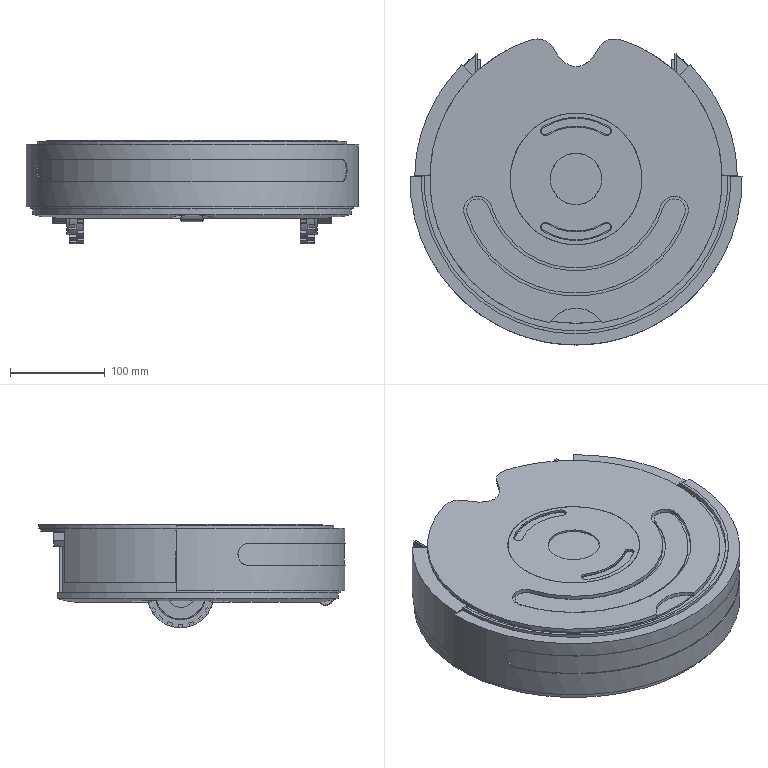Assembly | NX | mm | 13 component files | 13 solids | 690 faces | box 349.76 x 322.33 x 108.7 mm | volume 3327610 mm3 | plane 550 | cylinder 126 | cone 6 | other 5 | spline 3 | commonest cylinder face diameters 308 x6 30 x5 271.2 x4 8.023 x4 10.023 x4 52 x4 5 x4 336 x3
Bill of materials:
unnamed part 1 | 1 |  | Thick circular disc with two staggered rows of rectangular lugs around its outer rim, and a small cylindrical pin sticking out from the centre of one face.
unnamed part 2 | 1 |  | Curved, arc-shaped block segment with a stepped rectangular notch at one end, a thin raised pad on the top face, and a downward step projection.
unnamed part 3 | 1 |  | Thin flat round washer-like plate with a large central hole, two arc-shaped through-slots on opposite sides, and a small step around the outer edge.
unnamed part 4 | 1 |  | Thin flat round plate with an off-centre circular hole, one large arc-shaped through-slot, two rounded notches on opposite edges, and small tabs sticking out from one face.
unnamed part 5 | 1 |  | Lever- or cam-like part: a cylindrical arm with a rounded end joined to an offset, partly circular lobe that has a small through-hole.
unnamed part 6 | 1 |  | Thick circular disc with two staggered rows of rectangular lugs around its rim, a shallow concentric ring recess on one face, and a small cylindrical pin from the centre of that face.
unnamed part 7 | 1 |  | Rectangular block with a U-shaped profile: two upright end walls with stepped shoulders on either side of a lower central floor, and small rounded notches in the floor.
unnamed part 8 | 1 |  | Lever- or cam-like part: a cylindrical arm with a rounded end joined to an offset, partly circular lobe that has a small through-hole and a curved rim wall.
unnamed part 9 | 1 |  | Thin circular plate with a wide rectangular opening cut in from one edge, two rectangular windows near the sides of that opening, a circular hole near the opposite edge, low raised ribs, and a chamfered outer edge.
unnamed part 10 | 1 |  | Thick circular base with a rectangular notch cut from one side and several features on the top face: a raised concentric boss with a recess, curved ribs, and thin upright walls along the notch edges.
unnamed part 11 | 1 |  | Round annular plate with a large central hole, a rounded notch in the edge, two rectangular windows, a small slot, a raised concentric ring step, and a curved wall segment hanging down from part of the rim.
unnamed part 12 | 1 |  | Round flat disc head with a short cylindrical peg underneath, set with its axis lying parallel to the disc face; both have chamfered edges.
unnamed part 13 | 1 |  | Thin-walled semicircular (half-ring) shell: a 180-degree arc of constant radial thickness with flat end faces, an axial height several times the wall thickness, a narrow stepped band along one axial edge, a faint line around the outer surface, and small rounded slot-like recesses near the ends.
Mates:
1. concentric | Top_Cover 1 edge | Outer_Shell 1 edge
2. concentric | Inner_Shell 1 edge | Outer_Shell 1 edge
3. concentric | Front_Baffle 1 edge | Outer_Shell 1 edge
4. concentric | Baffle 1 edge | Inner_Shell 1 edge
5. concentric | Wheel_Mount 1 edge | Inner_Shell 1 edge
6. fix | Top_Cover 1 component
7. touch align | Wheel_Bracket 1 face | Wheel_Mount 1 face
8. distance | Inner_Shell 1 face | Wheel_Bracket 1 face
9. distance | Inner_Shell 1 face | Wheel_Bracket 1 face
10. concentric | Wheel 1 | Wheel_Bracket 1 edge
11. concentric | Front_Wheel 1 edge | Inner_Shell 1 edge
12. concentric | Bottom_Shell 1 edge | Inner_Shell 1 edge
13. center | Hopper 1 face | Hopper 1 face | Inner_Shell 1 face | Inner_Shell 1 face
14. touch align | Hopper 1 face | Inner_Shell 1 face
15. touch align | Hopper 1 face | Inner_Shell 1 face